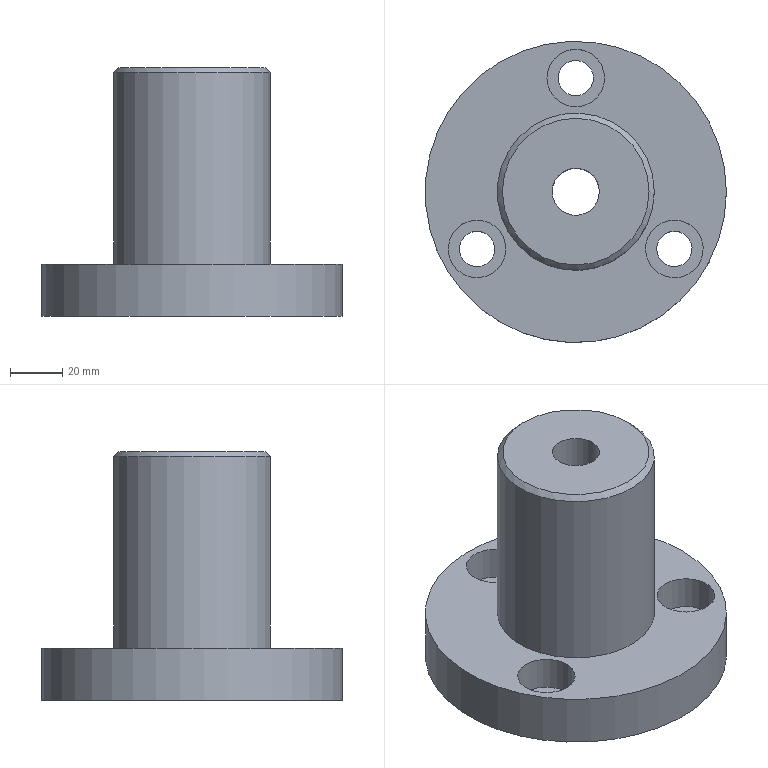Component | NX | DIE_SHANK | 1 solid | 16 faces | box 115 x 115 x 95 mm | volume 377421 mm3 | cylinder 9 | plane 6 | cone 1 | commonest cylinder face diameters 22 x3 13.5 x3 115 x1 60 x1 18 x1
STEP:
#1=CARTESIAN_POINT('',(0.,0.,0.));
#2=DIRECTION('',(0.,0.,1.));
#3=DIRECTION('',(1.,0.,0.));
#4=AXIS2_PLACEMENT_3D('',#1,#2,#3);
#5=CARTESIAN_POINT('',(43.172,-19.724,237.));
#6=VERTEX_POINT('',#5);
#7=CARTESIAN_POINT('',(37.672,-29.25,237.));
#8=DIRECTION('',(0.,0.,1.));
#9=DIRECTION('',(0.5,0.866,0.));
#10=AXIS2_PLACEMENT_3D('',#7,#8,#9);
#11=CIRCLE('',#10,11.);
#12=CARTESIAN_POINT('',(37.672,-29.25,250.));
#13=DIRECTION('',(0.,0.,-1.));
#14=DIRECTION('',(0.5,0.866,0.));
#15=AXIS2_PLACEMENT_3D('',#12,#13,#14);
#16=CYLINDRICAL_SURFACE('',#15,11.);
#17=CARTESIAN_POINT('',(6.283,13.));
#18=DIRECTION('',(-1.,0.));
#19=VECTOR('',#18,1.);
#20=LINE('',#17,#19);
#21=(GEOMETRIC_REPRESENTATION_CONTEXT(2)PARAMETRIC_REPRESENTATION_CONTEXT()REPRESENTATION_CONTEXT('',''));
#22=DEFINITIONAL_REPRESENTATION('',(#20),#21);
#23=PCURVE('',#16,#22);
#24=CARTESIAN_POINT('',(37.672,-29.25,237.));
#25=DIRECTION('',(0.,0.,-1.));
#26=DIRECTION('',(0.5,0.866,0.));
#27=AXIS2_PLACEMENT_3D('',#24,#25,#26);
#28=PLANE('',#27);
#29=CARTESIAN_POINT('',(11.,0.));
#30=CARTESIAN_POINT('',(11.,-19.053));
#31=CARTESIAN_POINT('',(-5.5,-9.526));
#32=CARTESIAN_POINT('',(-22.,-0.));
#33=CARTESIAN_POINT('',(-5.5,9.526));
#34=CARTESIAN_POINT('',(11.,19.053));
#35=CARTESIAN_POINT('',(11.,0.));
#36=(BOUNDED_CURVE()B_SPLINE_CURVE(2,(#29,#30,#31,#32,#33,#34,#35),.UNSPECIFIED.,.T.,.F.)B_SPLINE_CURVE_WITH_KNOTS((1,2,2,2,2,1),(-2.094,0.,2.094,4.189,6.283,8.378),.UNSPECIFIED.)CURVE()GEOMETRIC_REPRESENTATION_ITEM()RATIONAL_B_SPLINE_CURVE((1.,0.5,1.,0.5,1.,0.5,1.))REPRESENTATION_ITEM(''));
#37=(GEOMETRIC_REPRESENTATION_CONTEXT(2)PARAMETRIC_REPRESENTATION_CONTEXT()REPRESENTATION_CONTEXT('',''));
#38=DEFINITIONAL_REPRESENTATION('',(#36),#37);
#39=PCURVE('',#28,#38);
#40=SURFACE_CURVE('',#11,(#23,#39),.PCURVE_S1.);
#41=EDGE_CURVE('',#6,#6,#40,.T.);
#42=ORIENTED_EDGE('',*,*,#41,.T.);
#43=CARTESIAN_POINT('',(43.172,-19.724,250.));
#44=VERTEX_POINT('',#43);
#45=CARTESIAN_POINT('',(43.172,-19.724,250.));
#46=CARTESIAN_POINT('',(43.172,-19.724,237.));
#47=B_SPLINE_CURVE_WITH_KNOTS('',1,(#45,#46),.UNSPECIFIED.,.F.,.F.,(2,2),(0.,13.),.PIECEWISE_BEZIER_KNOTS.);
#48=CARTESIAN_POINT('',(0.,0.));
#49=DIRECTION('',(0.,1.));
#50=VECTOR('',#49,1.);
#51=LINE('',#48,#50);
#52=(GEOMETRIC_REPRESENTATION_CONTEXT(2)PARAMETRIC_REPRESENTATION_CONTEXT()REPRESENTATION_CONTEXT('',''));
#53=DEFINITIONAL_REPRESENTATION('',(#51),#52);
#54=PCURVE('',#16,#53);
#55=CARTESIAN_POINT('',(6.283,0.));
#56=DIRECTION('',(0.,1.));
#57=VECTOR('',#56,1.);
#58=LINE('',#55,#57);
#59=(GEOMETRIC_REPRESENTATION_CONTEXT(2)PARAMETRIC_REPRESENTATION_CONTEXT()REPRESENTATION_CONTEXT('',''));
#60=DEFINITIONAL_REPRESENTATION('',(#58),#59);
#61=PCURVE('',#16,#60);
#62=SEAM_CURVE('',#47,(#54,#61),.PCURVE_S1.);
#63=EDGE_CURVE('',#44,#6,#62,.T.);
#64=ORIENTED_EDGE('',*,*,#63,.F.);
#65=CARTESIAN_POINT('',(37.672,-29.25,250.));
#66=DIRECTION('',(0.,0.,-1.));
#67=DIRECTION('',(0.5,0.866,0.));
#68=AXIS2_PLACEMENT_3D('',#65,#66,#67);
#69=CIRCLE('',#68,11.);
#70=CARTESIAN_POINT('',(0.,0.));
#71=DIRECTION('',(1.,0.));
#72=VECTOR('',#71,1.);
#73=LINE('',#70,#72);
#74=(GEOMETRIC_REPRESENTATION_CONTEXT(2)PARAMETRIC_REPRESENTATION_CONTEXT()REPRESENTATION_CONTEXT('',''));
#75=DEFINITIONAL_REPRESENTATION('',(#73),#74);
#76=PCURVE('',#16,#75);
#77=CARTESIAN_POINT('',(-0.,-7.5,250.));
#78=DIRECTION('',(0.,0.,1.));
#79=DIRECTION('',(1.,0.,0.));
#80=AXIS2_PLACEMENT_3D('',#77,#78,#79);
#81=PLANE('',#80);
#82=CARTESIAN_POINT('',(43.172,-12.224));
#83=CARTESIAN_POINT('',(59.672,-21.75));
#84=CARTESIAN_POINT('',(43.172,-31.276));
#85=CARTESIAN_POINT('',(26.672,-40.803));
#86=CARTESIAN_POINT('',(26.672,-21.75));
#87=CARTESIAN_POINT('',(26.672,-2.697));
#88=CARTESIAN_POINT('',(43.172,-12.224));
#89=(BOUNDED_CURVE()B_SPLINE_CURVE(2,(#82,#83,#84,#85,#86,#87,#88),.UNSPECIFIED.,.T.,.F.)B_SPLINE_CURVE_WITH_KNOTS((1,2,2,2,2,1),(-2.094,0.,2.094,4.189,6.283,8.378),.UNSPECIFIED.)CURVE()GEOMETRIC_REPRESENTATION_ITEM()RATIONAL_B_SPLINE_CURVE((1.,0.5,1.,0.5,1.,0.5,1.))REPRESENTATION_ITEM(''));
#90=(GEOMETRIC_REPRESENTATION_CONTEXT(2)PARAMETRIC_REPRESENTATION_CONTEXT()REPRESENTATION_CONTEXT('',''));
#91=DEFINITIONAL_REPRESENTATION('',(#89),#90);
#92=PCURVE('',#81,#91);
#93=SURFACE_CURVE('',#69,(#76,#92),.PCURVE_S1.);
#94=EDGE_CURVE('',#44,#44,#93,.T.);
#95=ORIENTED_EDGE('',*,*,#94,.T.);
#96=ORIENTED_EDGE('',*,*,#63,.T.);
#97=EDGE_LOOP('',(#42,#64,#95,#96));
#98=FACE_BOUND('',#97,.F.);
#99=ADVANCED_FACE('',(#98),#16,.F.);
#100=CARTESIAN_POINT('',(41.047,-23.404,237.));
#101=VERTEX_POINT('',#100);
#102=CARTESIAN_POINT('',(37.672,-29.25,237.));
#103=DIRECTION('',(0.,0.,1.));
#104=DIRECTION('',(0.5,0.866,0.));
#105=AXIS2_PLACEMENT_3D('',#102,#103,#104);
#106=CIRCLE('',#105,6.75);
#107=CARTESIAN_POINT('',(6.75,0.));
#108=CARTESIAN_POINT('',(6.75,-11.691));
#109=CARTESIAN_POINT('',(-3.375,-5.846));
#110=CARTESIAN_POINT('',(-13.5,-0.));
#111=CARTESIAN_POINT('',(-3.375,5.846));
#112=CARTESIAN_POINT('',(6.75,11.691));
#113=CARTESIAN_POINT('',(6.75,0.));
#114=(BOUNDED_CURVE()B_SPLINE_CURVE(2,(#107,#108,#109,#110,#111,#112,#113),.UNSPECIFIED.,.T.,.F.)B_SPLINE_CURVE_WITH_KNOTS((1,2,2,2,2,1),(-2.094,0.,2.094,4.189,6.283,8.378),.UNSPECIFIED.)CURVE()GEOMETRIC_REPRESENTATION_ITEM()RATIONAL_B_SPLINE_CURVE((1.,0.5,1.,0.5,1.,0.5,1.))REPRESENTATION_ITEM(''));
#115=(GEOMETRIC_REPRESENTATION_CONTEXT(2)PARAMETRIC_REPRESENTATION_CONTEXT()REPRESENTATION_CONTEXT('',''));
#116=DEFINITIONAL_REPRESENTATION('',(#114),#115);
#117=PCURVE('',#28,#116);
#118=CARTESIAN_POINT('',(37.672,-29.25,183.484));
#119=DIRECTION('',(0.,0.,-1.));
#120=DIRECTION('',(0.5,0.866,0.));
#121=AXIS2_PLACEMENT_3D('',#118,#119,#120);
#122=CYLINDRICAL_SURFACE('',#121,6.75);
#123=CARTESIAN_POINT('',(6.283,-53.516));
#124=DIRECTION('',(-1.,0.));
#125=VECTOR('',#124,1.);
#126=LINE('',#123,#125);
#127=(GEOMETRIC_REPRESENTATION_CONTEXT(2)PARAMETRIC_REPRESENTATION_CONTEXT()REPRESENTATION_CONTEXT('',''));
#128=DEFINITIONAL_REPRESENTATION('',(#126),#127);
#129=PCURVE('',#122,#128);
#130=SURFACE_CURVE('',#106,(#117,#129),.PCURVE_S1.);
#131=EDGE_CURVE('',#101,#101,#130,.T.);
#132=ORIENTED_EDGE('',*,*,#131,.F.);
#133=EDGE_LOOP('',(#132));
#134=FACE_BOUND('',#133,.T.);
#135=ORIENTED_EDGE('',*,*,#41,.T.);
#136=EDGE_LOOP('',(#135));
#137=FACE_BOUND('',#136,.T.);
#138=ADVANCED_FACE('',(#134,#137),#28,.F.);
#139=CARTESIAN_POINT('',(41.047,-23.404,230.));
#140=VERTEX_POINT('',#139);
#141=CARTESIAN_POINT('',(37.672,-29.25,230.));
#142=DIRECTION('',(0.,0.,-1.));
#143=DIRECTION('',(0.5,0.866,0.));
#144=AXIS2_PLACEMENT_3D('',#141,#142,#143);
#145=CIRCLE('',#144,6.75);
#146=CARTESIAN_POINT('',(0.,-46.516));
#147=DIRECTION('',(1.,0.));
#148=VECTOR('',#147,1.);
#149=LINE('',#146,#148);
#150=(GEOMETRIC_REPRESENTATION_CONTEXT(2)PARAMETRIC_REPRESENTATION_CONTEXT()REPRESENTATION_CONTEXT('',''));
#151=DEFINITIONAL_REPRESENTATION('',(#149),#150);
#152=PCURVE('',#122,#151);
#153=CARTESIAN_POINT('',(-0.,-7.5,230.));
#154=DIRECTION('',(0.,0.,-1.));
#155=DIRECTION('',(-1.,0.,0.));
#156=AXIS2_PLACEMENT_3D('',#153,#154,#155);
#157=PLANE('',#156);
#158=CARTESIAN_POINT('',(-37.672,-21.75));
#159=DIRECTION('',(-0.5,0.866));
#160=AXIS2_PLACEMENT_2D('',#158,#159);
#161=CIRCLE('',#160,6.75);
#162=(GEOMETRIC_REPRESENTATION_CONTEXT(2)PARAMETRIC_REPRESENTATION_CONTEXT()REPRESENTATION_CONTEXT('',''));
#163=DEFINITIONAL_REPRESENTATION('',(#161),#162);
#164=PCURVE('',#157,#163);
#165=SURFACE_CURVE('',#145,(#152,#164),.PCURVE_S1.);
#166=EDGE_CURVE('',#140,#140,#165,.T.);
#167=ORIENTED_EDGE('',*,*,#166,.F.);
#168=CARTESIAN_POINT('',(41.047,-23.404,237.));
#169=CARTESIAN_POINT('',(41.047,-23.404,230.));
#170=B_SPLINE_CURVE_WITH_KNOTS('',1,(#168,#169),.UNSPECIFIED.,.F.,.F.,(2,2),(-53.516,-46.516),.PIECEWISE_BEZIER_KNOTS.);
#171=CARTESIAN_POINT('',(0.,0.));
#172=DIRECTION('',(0.,1.));
#173=VECTOR('',#172,1.);
#174=LINE('',#171,#173);
#175=(GEOMETRIC_REPRESENTATION_CONTEXT(2)PARAMETRIC_REPRESENTATION_CONTEXT()REPRESENTATION_CONTEXT('',''));
#176=DEFINITIONAL_REPRESENTATION('',(#174),#175);
#177=PCURVE('',#122,#176);
#178=CARTESIAN_POINT('',(6.283,0.));
#179=DIRECTION('',(0.,1.));
#180=VECTOR('',#179,1.);
#181=LINE('',#178,#180);
#182=(GEOMETRIC_REPRESENTATION_CONTEXT(2)PARAMETRIC_REPRESENTATION_CONTEXT()REPRESENTATION_CONTEXT('',''));
#183=DEFINITIONAL_REPRESENTATION('',(#181),#182);
#184=PCURVE('',#122,#183);
#185=SEAM_CURVE('',#170,(#177,#184),.PCURVE_S1.);
#186=EDGE_CURVE('',#101,#140,#185,.T.);
#187=ORIENTED_EDGE('',*,*,#186,.F.);
#188=ORIENTED_EDGE('',*,*,#131,.F.);
#189=ORIENTED_EDGE('',*,*,#186,.T.);
#190=EDGE_LOOP('',(#167,#187,#188,#189));
#191=FACE_BOUND('',#190,.F.);
#192=ADVANCED_FACE('',(#191),#122,.F.);
#193=CARTESIAN_POINT('',(-32.172,-38.776,237.));
#194=VERTEX_POINT('',#193);
#195=CARTESIAN_POINT('',(-37.672,-29.25,237.));
#196=DIRECTION('',(0.,0.,1.));
#197=DIRECTION('',(0.5,-0.866,0.));
#198=AXIS2_PLACEMENT_3D('',#195,#196,#197);
#199=CIRCLE('',#198,11.);
#200=CARTESIAN_POINT('',(-37.672,-29.25,250.));
#201=DIRECTION('',(0.,0.,-1.));
#202=DIRECTION('',(0.5,-0.866,0.));
#203=AXIS2_PLACEMENT_3D('',#200,#201,#202);
#204=CYLINDRICAL_SURFACE('',#203,11.);
#205=CARTESIAN_POINT('',(6.283,13.));
#206=DIRECTION('',(-1.,0.));
#207=VECTOR('',#206,1.);
#208=LINE('',#205,#207);
#209=(GEOMETRIC_REPRESENTATION_CONTEXT(2)PARAMETRIC_REPRESENTATION_CONTEXT()REPRESENTATION_CONTEXT('',''));
#210=DEFINITIONAL_REPRESENTATION('',(#208),#209);
#211=PCURVE('',#204,#210);
#212=CARTESIAN_POINT('',(-37.672,-29.25,237.));
#213=DIRECTION('',(0.,0.,-1.));
#214=DIRECTION('',(0.5,-0.866,0.));
#215=AXIS2_PLACEMENT_3D('',#212,#213,#214);
#216=PLANE('',#215);
#217=CARTESIAN_POINT('',(11.,0.));
#218=CARTESIAN_POINT('',(11.,-19.053));
#219=CARTESIAN_POINT('',(-5.5,-9.526));
#220=CARTESIAN_POINT('',(-22.,-0.));
#221=CARTESIAN_POINT('',(-5.5,9.526));
#222=CARTESIAN_POINT('',(11.,19.053));
#223=CARTESIAN_POINT('',(11.,0.));
#224=(BOUNDED_CURVE()B_SPLINE_CURVE(2,(#217,#218,#219,#220,#221,#222,#223),.UNSPECIFIED.,.T.,.F.)B_SPLINE_CURVE_WITH_KNOTS((1,2,2,2,2,1),(-2.094,0.,2.094,4.189,6.283,8.378),.UNSPECIFIED.)CURVE()GEOMETRIC_REPRESENTATION_ITEM()RATIONAL_B_SPLINE_CURVE((1.,0.5,1.,0.5,1.,0.5,1.))REPRESENTATION_ITEM(''));
#225=(GEOMETRIC_REPRESENTATION_CONTEXT(2)PARAMETRIC_REPRESENTATION_CONTEXT()REPRESENTATION_CONTEXT('',''));
#226=DEFINITIONAL_REPRESENTATION('',(#224),#225);
#227=PCURVE('',#216,#226);
#228=SURFACE_CURVE('',#199,(#211,#227),.PCURVE_S1.);
#229=EDGE_CURVE('',#194,#194,#228,.T.);
#230=ORIENTED_EDGE('',*,*,#229,.T.);
#231=CARTESIAN_POINT('',(-32.172,-38.776,250.));
#232=VERTEX_POINT('',#231);
#233=CARTESIAN_POINT('',(-32.172,-38.776,250.));
#234=CARTESIAN_POINT('',(-32.172,-38.776,237.));
#235=B_SPLINE_CURVE_WITH_KNOTS('',1,(#233,#234),.UNSPECIFIED.,.F.,.F.,(2,2),(0.,13.),.PIECEWISE_BEZIER_KNOTS.);
#236=CARTESIAN_POINT('',(0.,0.));
#237=DIRECTION('',(0.,1.));
#238=VECTOR('',#237,1.);
#239=LINE('',#236,#238);
#240=(GEOMETRIC_REPRESENTATION_CONTEXT(2)PARAMETRIC_REPRESENTATION_CONTEXT()REPRESENTATION_CONTEXT('',''));
#241=DEFINITIONAL_REPRESENTATION('',(#239),#240);
#242=PCURVE('',#204,#241);
#243=CARTESIAN_POINT('',(6.283,0.));
#244=DIRECTION('',(0.,1.));
#245=VECTOR('',#244,1.);
#246=LINE('',#243,#245);
#247=(GEOMETRIC_REPRESENTATION_CONTEXT(2)PARAMETRIC_REPRESENTATION_CONTEXT()REPRESENTATION_CONTEXT('',''));
#248=DEFINITIONAL_REPRESENTATION('',(#246),#247);
#249=PCURVE('',#204,#248);
#250=SEAM_CURVE('',#235,(#242,#249),.PCURVE_S1.);
#251=EDGE_CURVE('',#232,#194,#250,.T.);
#252=ORIENTED_EDGE('',*,*,#251,.F.);
#253=CARTESIAN_POINT('',(-37.672,-29.25,250.));
#254=DIRECTION('',(0.,0.,-1.));
#255=DIRECTION('',(0.5,-0.866,0.));
#256=AXIS2_PLACEMENT_3D('',#253,#254,#255);
#257=CIRCLE('',#256,11.);
#258=CARTESIAN_POINT('',(0.,0.));
#259=DIRECTION('',(1.,0.));
#260=VECTOR('',#259,1.);
#261=LINE('',#258,#260);
#262=(GEOMETRIC_REPRESENTATION_CONTEXT(2)PARAMETRIC_REPRESENTATION_CONTEXT()REPRESENTATION_CONTEXT('',''));
#263=DEFINITIONAL_REPRESENTATION('',(#261),#262);
#264=PCURVE('',#204,#263);
#265=CARTESIAN_POINT('',(-32.172,-31.276));
#266=CARTESIAN_POINT('',(-48.672,-40.803));
#267=CARTESIAN_POINT('',(-48.672,-21.75));
#268=CARTESIAN_POINT('',(-48.672,-2.697));
#269=CARTESIAN_POINT('',(-32.172,-12.224));
#270=CARTESIAN_POINT('',(-15.672,-21.75));
#271=CARTESIAN_POINT('',(-32.172,-31.276));
#272=(BOUNDED_CURVE()B_SPLINE_CURVE(2,(#265,#266,#267,#268,#269,#270,#271),.UNSPECIFIED.,.T.,.F.)B_SPLINE_CURVE_WITH_KNOTS((1,2,2,2,2,1),(-2.094,0.,2.094,4.189,6.283,8.378),.UNSPECIFIED.)CURVE()GEOMETRIC_REPRESENTATION_ITEM()RATIONAL_B_SPLINE_CURVE((1.,0.5,1.,0.5,1.,0.5,1.))REPRESENTATION_ITEM(''));
#273=(GEOMETRIC_REPRESENTATION_CONTEXT(2)PARAMETRIC_REPRESENTATION_CONTEXT()REPRESENTATION_CONTEXT('',''));
#274=DEFINITIONAL_REPRESENTATION('',(#272),#273);
#275=PCURVE('',#81,#274);
#276=SURFACE_CURVE('',#257,(#264,#275),.PCURVE_S1.);
#277=EDGE_CURVE('',#232,#232,#276,.T.);
#278=ORIENTED_EDGE('',*,*,#277,.T.);
#279=ORIENTED_EDGE('',*,*,#251,.T.);
#280=EDGE_LOOP('',(#230,#252,#278,#279));
#281=FACE_BOUND('',#280,.F.);
#282=ADVANCED_FACE('',(#281),#204,.F.);
#283=CARTESIAN_POINT('',(-34.297,-35.096,237.));
#284=VERTEX_POINT('',#283);
#285=CARTESIAN_POINT('',(-37.672,-29.25,237.));
#286=DIRECTION('',(0.,0.,1.));
#287=DIRECTION('',(0.5,-0.866,0.));
#288=AXIS2_PLACEMENT_3D('',#285,#286,#287);
#289=CIRCLE('',#288,6.75);
#290=CARTESIAN_POINT('',(6.75,0.));
#291=CARTESIAN_POINT('',(6.75,-11.691));
#292=CARTESIAN_POINT('',(-3.375,-5.846));
#293=CARTESIAN_POINT('',(-13.5,-0.));
#294=CARTESIAN_POINT('',(-3.375,5.846));
#295=CARTESIAN_POINT('',(6.75,11.691));
#296=CARTESIAN_POINT('',(6.75,0.));
#297=(BOUNDED_CURVE()B_SPLINE_CURVE(2,(#290,#291,#292,#293,#294,#295,#296),.UNSPECIFIED.,.T.,.F.)B_SPLINE_CURVE_WITH_KNOTS((1,2,2,2,2,1),(-2.094,0.,2.094,4.189,6.283,8.378),.UNSPECIFIED.)CURVE()GEOMETRIC_REPRESENTATION_ITEM()RATIONAL_B_SPLINE_CURVE((1.,0.5,1.,0.5,1.,0.5,1.))REPRESENTATION_ITEM(''));
#298=(GEOMETRIC_REPRESENTATION_CONTEXT(2)PARAMETRIC_REPRESENTATION_CONTEXT()REPRESENTATION_CONTEXT('',''));
#299=DEFINITIONAL_REPRESENTATION('',(#297),#298);
#300=PCURVE('',#216,#299);
#301=CARTESIAN_POINT('',(-37.672,-29.25,183.484));
#302=DIRECTION('',(0.,0.,-1.));
#303=DIRECTION('',(0.5,-0.866,0.));
#304=AXIS2_PLACEMENT_3D('',#301,#302,#303);
#305=CYLINDRICAL_SURFACE('',#304,6.75);
#306=CARTESIAN_POINT('',(6.283,-53.516));
#307=DIRECTION('',(-1.,0.));
#308=VECTOR('',#307,1.);
#309=LINE('',#306,#308);
#310=(GEOMETRIC_REPRESENTATION_CONTEXT(2)PARAMETRIC_REPRESENTATION_CONTEXT()REPRESENTATION_CONTEXT('',''));
#311=DEFINITIONAL_REPRESENTATION('',(#309),#310);
#312=PCURVE('',#305,#311);
#313=SURFACE_CURVE('',#289,(#300,#312),.PCURVE_S1.);
#314=EDGE_CURVE('',#284,#284,#313,.T.);
#315=ORIENTED_EDGE('',*,*,#314,.F.);
#316=EDGE_LOOP('',(#315));
#317=FACE_BOUND('',#316,.T.);
#318=ORIENTED_EDGE('',*,*,#229,.T.);
#319=EDGE_LOOP('',(#318));
#320=FACE_BOUND('',#319,.T.);
#321=ADVANCED_FACE('',(#317,#320),#216,.F.);
#322=CARTESIAN_POINT('',(-34.297,-35.096,230.));
#323=VERTEX_POINT('',#322);
#324=CARTESIAN_POINT('',(-37.672,-29.25,230.));
#325=DIRECTION('',(0.,0.,-1.));
#326=DIRECTION('',(0.5,-0.866,0.));
#327=AXIS2_PLACEMENT_3D('',#324,#325,#326);
#328=CIRCLE('',#327,6.75);
#329=CARTESIAN_POINT('',(0.,-46.516));
#330=DIRECTION('',(1.,0.));
#331=VECTOR('',#330,1.);
#332=LINE('',#329,#331);
#333=(GEOMETRIC_REPRESENTATION_CONTEXT(2)PARAMETRIC_REPRESENTATION_CONTEXT()REPRESENTATION_CONTEXT('',''));
#334=DEFINITIONAL_REPRESENTATION('',(#332),#333);
#335=PCURVE('',#305,#334);
#336=CARTESIAN_POINT('',(37.672,-21.75));
#337=DIRECTION('',(-0.5,-0.866));
#338=AXIS2_PLACEMENT_2D('',#336,#337);
#339=CIRCLE('',#338,6.75);
#340=(GEOMETRIC_REPRESENTATION_CONTEXT(2)PARAMETRIC_REPRESENTATION_CONTEXT()REPRESENTATION_CONTEXT('',''));
#341=DEFINITIONAL_REPRESENTATION('',(#339),#340);
#342=PCURVE('',#157,#341);
#343=SURFACE_CURVE('',#328,(#335,#342),.PCURVE_S1.);
#344=EDGE_CURVE('',#323,#323,#343,.T.);
#345=ORIENTED_EDGE('',*,*,#344,.F.);
#346=CARTESIAN_POINT('',(-34.297,-35.096,237.));
#347=CARTESIAN_POINT('',(-34.297,-35.096,230.));
#348=B_SPLINE_CURVE_WITH_KNOTS('',1,(#346,#347),.UNSPECIFIED.,.F.,.F.,(2,2),(-53.516,-46.516),.PIECEWISE_BEZIER_KNOTS.);
#349=CARTESIAN_POINT('',(0.,0.));
#350=DIRECTION('',(0.,1.));
#351=VECTOR('',#350,1.);
#352=LINE('',#349,#351);
#353=(GEOMETRIC_REPRESENTATION_CONTEXT(2)PARAMETRIC_REPRESENTATION_CONTEXT()REPRESENTATION_CONTEXT('',''));
#354=DEFINITIONAL_REPRESENTATION('',(#352),#353);
#355=PCURVE('',#305,#354);
#356=CARTESIAN_POINT('',(6.283,0.));
#357=DIRECTION('',(0.,1.));
#358=VECTOR('',#357,1.);
#359=LINE('',#356,#358);
#360=(GEOMETRIC_REPRESENTATION_CONTEXT(2)PARAMETRIC_REPRESENTATION_CONTEXT()REPRESENTATION_CONTEXT('',''));
#361=DEFINITIONAL_REPRESENTATION('',(#359),#360);
#362=PCURVE('',#305,#361);
#363=SEAM_CURVE('',#348,(#355,#362),.PCURVE_S1.);
#364=EDGE_CURVE('',#284,#323,#363,.T.);
#365=ORIENTED_EDGE('',*,*,#364,.F.);
#366=ORIENTED_EDGE('',*,*,#314,.F.);
#367=ORIENTED_EDGE('',*,*,#364,.T.);
#368=EDGE_LOOP('',(#345,#365,#366,#367));
#369=FACE_BOUND('',#368,.F.);
#370=ADVANCED_FACE('',(#369),#305,.F.);
#371=ORIENTED_EDGE('',*,*,#94,.T.);
#372=EDGE_LOOP('',(#371));
#373=FACE_BOUND('',#372,.T.);
#374=ORIENTED_EDGE('',*,*,#277,.T.);
#375=EDGE_LOOP('',(#374));
#376=FACE_BOUND('',#375,.T.);
#377=CARTESIAN_POINT('',(-11.,36.,250.));
#378=VERTEX_POINT('',#377);
#379=CARTESIAN_POINT('',(-0.,36.,250.));
#380=DIRECTION('',(0.,0.,-1.));
#381=DIRECTION('',(-1.,0.,0.));
#382=AXIS2_PLACEMENT_3D('',#379,#380,#381);
#383=CIRCLE('',#382,11.);
#384=CARTESIAN_POINT('',(-11.,43.5));
#385=CARTESIAN_POINT('',(-11.,62.553));
#386=CARTESIAN_POINT('',(5.5,53.026));
#387=CARTESIAN_POINT('',(22.,43.5));
#388=CARTESIAN_POINT('',(5.5,33.974));
#389=CARTESIAN_POINT('',(-11.,24.447));
#390=CARTESIAN_POINT('',(-11.,43.5));
#391=(BOUNDED_CURVE()B_SPLINE_CURVE(2,(#384,#385,#386,#387,#388,#389,#390),.UNSPECIFIED.,.T.,.F.)B_SPLINE_CURVE_WITH_KNOTS((1,2,2,2,2,1),(-2.094,0.,2.094,4.189,6.283,8.378),.UNSPECIFIED.)CURVE()GEOMETRIC_REPRESENTATION_ITEM()RATIONAL_B_SPLINE_CURVE((1.,0.5,1.,0.5,1.,0.5,1.))REPRESENTATION_ITEM(''));
#392=(GEOMETRIC_REPRESENTATION_CONTEXT(2)PARAMETRIC_REPRESENTATION_CONTEXT()REPRESENTATION_CONTEXT('',''));
#393=DEFINITIONAL_REPRESENTATION('',(#391),#392);
#394=PCURVE('',#81,#393);
#395=CARTESIAN_POINT('',(-0.,36.,250.));
#396=DIRECTION('',(0.,0.,-1.));
#397=DIRECTION('',(-1.,0.,0.));
#398=AXIS2_PLACEMENT_3D('',#395,#396,#397);
#399=CYLINDRICAL_SURFACE('',#398,11.);
#400=CARTESIAN_POINT('',(0.,0.));
#401=DIRECTION('',(1.,0.));
#402=VECTOR('',#401,1.);
#403=LINE('',#400,#402);
#404=(GEOMETRIC_REPRESENTATION_CONTEXT(2)PARAMETRIC_REPRESENTATION_CONTEXT()REPRESENTATION_CONTEXT('',''));
#405=DEFINITIONAL_REPRESENTATION('',(#403),#404);
#406=PCURVE('',#399,#405);
#407=SURFACE_CURVE('',#383,(#394,#406),.PCURVE_S1.);
#408=EDGE_CURVE('',#378,#378,#407,.T.);
#409=ORIENTED_EDGE('',*,*,#408,.T.);
#410=EDGE_LOOP('',(#409));
#411=FACE_BOUND('',#410,.T.);
#412=CARTESIAN_POINT('',(30.,-7.5,250.));
#413=VERTEX_POINT('',#412);
#414=CARTESIAN_POINT('',(-0.,-7.5,250.));
#415=DIRECTION('',(0.,0.,1.));
#416=DIRECTION('',(1.,0.,0.));
#417=AXIS2_PLACEMENT_3D('',#414,#415,#416);
#418=CIRCLE('',#417,30.);
#419=CARTESIAN_POINT('',(0.,0.));
#420=DIRECTION('',(1.,0.));
#421=AXIS2_PLACEMENT_2D('',#419,#420);
#422=CIRCLE('',#421,30.);
#423=(GEOMETRIC_REPRESENTATION_CONTEXT(2)PARAMETRIC_REPRESENTATION_CONTEXT()REPRESENTATION_CONTEXT('',''));
#424=DEFINITIONAL_REPRESENTATION('',(#422),#423);
#425=PCURVE('',#81,#424);
#426=CARTESIAN_POINT('',(-0.,-7.5,250.));
#427=DIRECTION('',(0.,0.,1.));
#428=DIRECTION('',(1.,0.,0.));
#429=AXIS2_PLACEMENT_3D('',#426,#427,#428);
#430=CYLINDRICAL_SURFACE('',#429,30.);
#431=CARTESIAN_POINT('',(0.,0.));
#432=DIRECTION('',(1.,0.));
#433=VECTOR('',#432,1.);
#434=LINE('',#431,#433);
#435=(GEOMETRIC_REPRESENTATION_CONTEXT(2)PARAMETRIC_REPRESENTATION_CONTEXT()REPRESENTATION_CONTEXT('',''));
#436=DEFINITIONAL_REPRESENTATION('',(#434),#435);
#437=PCURVE('',#430,#436);
#438=SURFACE_CURVE('',#418,(#425,#437),.PCURVE_S1.);
#439=EDGE_CURVE('',#413,#413,#438,.T.);
#440=ORIENTED_EDGE('',*,*,#439,.F.);
#441=EDGE_LOOP('',(#440));
#442=FACE_BOUND('',#441,.T.);
#443=CARTESIAN_POINT('',(57.5,-7.5,250.));
#444=VERTEX_POINT('',#443);
#445=CARTESIAN_POINT('',(-0.,-7.5,250.));
#446=DIRECTION('',(0.,0.,-1.));
#447=DIRECTION('',(1.,0.,0.));
#448=AXIS2_PLACEMENT_3D('',#445,#446,#447);
#449=CIRCLE('',#448,57.5);
#450=CARTESIAN_POINT('',(57.5,0.));
#451=CARTESIAN_POINT('',(57.5,-99.593));
#452=CARTESIAN_POINT('',(-28.75,-49.796));
#453=CARTESIAN_POINT('',(-115.,-0.));
#454=CARTESIAN_POINT('',(-28.75,49.796));
#455=CARTESIAN_POINT('',(57.5,99.593));
#456=CARTESIAN_POINT('',(57.5,0.));
#457=(BOUNDED_CURVE()B_SPLINE_CURVE(2,(#450,#451,#452,#453,#454,#455,#456),.UNSPECIFIED.,.T.,.F.)B_SPLINE_CURVE_WITH_KNOTS((1,2,2,2,2,1),(-2.094,0.,2.094,4.189,6.283,8.378),.UNSPECIFIED.)CURVE()GEOMETRIC_REPRESENTATION_ITEM()RATIONAL_B_SPLINE_CURVE((1.,0.5,1.,0.5,1.,0.5,1.))REPRESENTATION_ITEM(''));
#458=(GEOMETRIC_REPRESENTATION_CONTEXT(2)PARAMETRIC_REPRESENTATION_CONTEXT()REPRESENTATION_CONTEXT('',''));
#459=DEFINITIONAL_REPRESENTATION('',(#457),#458);
#460=PCURVE('',#81,#459);
#461=CARTESIAN_POINT('',(-0.,-7.5,230.));
#462=DIRECTION('',(0.,0.,1.));
#463=DIRECTION('',(1.,0.,0.));
#464=AXIS2_PLACEMENT_3D('',#461,#462,#463);
#465=CYLINDRICAL_SURFACE('',#464,57.5);
#466=CARTESIAN_POINT('',(6.283,20.));
#467=DIRECTION('',(-1.,0.));
#468=VECTOR('',#467,1.);
#469=LINE('',#466,#468);
#470=(GEOMETRIC_REPRESENTATION_CONTEXT(2)PARAMETRIC_REPRESENTATION_CONTEXT()REPRESENTATION_CONTEXT('',''));
#471=DEFINITIONAL_REPRESENTATION('',(#469),#470);
#472=PCURVE('',#465,#471);
#473=SURFACE_CURVE('',#449,(#460,#472),.PCURVE_S1.);
#474=EDGE_CURVE('',#444,#444,#473,.T.);
#475=ORIENTED_EDGE('',*,*,#474,.F.);
#476=EDGE_LOOP('',(#475));
#477=FACE_BOUND('',#476,.T.);
#478=ADVANCED_FACE('',(#373,#376,#411,#442,#477),#81,.T.);
#479=ORIENTED_EDGE('',*,*,#166,.F.);
#480=EDGE_LOOP('',(#479));
#481=FACE_BOUND('',#480,.T.);
#482=ORIENTED_EDGE('',*,*,#344,.F.);
#483=EDGE_LOOP('',(#482));
#484=FACE_BOUND('',#483,.T.);
#485=CARTESIAN_POINT('',(-6.75,36.,230.));
#486=VERTEX_POINT('',#485);
#487=CARTESIAN_POINT('',(-0.,36.,230.));
#488=DIRECTION('',(0.,0.,-1.));
#489=DIRECTION('',(-1.,0.,0.));
#490=AXIS2_PLACEMENT_3D('',#487,#488,#489);
#491=CIRCLE('',#490,6.75);
#492=CARTESIAN_POINT('',(0.,43.5));
#493=DIRECTION('',(1.,0.));
#494=AXIS2_PLACEMENT_2D('',#492,#493);
#495=CIRCLE('',#494,6.75);
#496=(GEOMETRIC_REPRESENTATION_CONTEXT(2)PARAMETRIC_REPRESENTATION_CONTEXT()REPRESENTATION_CONTEXT('',''));
#497=DEFINITIONAL_REPRESENTATION('',(#495),#496);
#498=PCURVE('',#157,#497);
#499=CARTESIAN_POINT('',(-0.,36.,183.484));
#500=DIRECTION('',(0.,0.,-1.));
#501=DIRECTION('',(-1.,0.,0.));
#502=AXIS2_PLACEMENT_3D('',#499,#500,#501);
#503=CYLINDRICAL_SURFACE('',#502,6.75);
#504=CARTESIAN_POINT('',(0.,-46.516));
#505=DIRECTION('',(1.,0.));
#506=VECTOR('',#505,1.);
#507=LINE('',#504,#506);
#508=(GEOMETRIC_REPRESENTATION_CONTEXT(2)PARAMETRIC_REPRESENTATION_CONTEXT()REPRESENTATION_CONTEXT('',''));
#509=DEFINITIONAL_REPRESENTATION('',(#507),#508);
#510=PCURVE('',#503,#509);
#511=SURFACE_CURVE('',#491,(#498,#510),.PCURVE_S1.);
#512=EDGE_CURVE('',#486,#486,#511,.T.);
#513=ORIENTED_EDGE('',*,*,#512,.F.);
#514=EDGE_LOOP('',(#513));
#515=FACE_BOUND('',#514,.T.);
#516=CARTESIAN_POINT('',(-9.,-7.5,230.));
#517=VERTEX_POINT('',#516);
#518=CARTESIAN_POINT('',(-0.,-7.5,230.));
#519=DIRECTION('',(0.,0.,-1.));
#520=DIRECTION('',(-1.,0.,0.));
#521=AXIS2_PLACEMENT_3D('',#518,#519,#520);
#522=CIRCLE('',#521,9.);
#523=CARTESIAN_POINT('',(0.,0.));
#524=DIRECTION('',(1.,0.));
#525=AXIS2_PLACEMENT_2D('',#523,#524);
#526=CIRCLE('',#525,9.);
#527=(GEOMETRIC_REPRESENTATION_CONTEXT(2)PARAMETRIC_REPRESENTATION_CONTEXT()REPRESENTATION_CONTEXT('',''));
#528=DEFINITIONAL_REPRESENTATION('',(#526),#527);
#529=PCURVE('',#157,#528);
#530=CARTESIAN_POINT('',(-0.,-7.5,325.));
#531=DIRECTION('',(0.,0.,-1.));
#532=DIRECTION('',(-1.,0.,0.));
#533=AXIS2_PLACEMENT_3D('',#530,#531,#532);
#534=CYLINDRICAL_SURFACE('',#533,9.);
#535=CARTESIAN_POINT('',(0.,95.));
#536=DIRECTION('',(1.,0.));
#537=VECTOR('',#536,1.);
#538=LINE('',#535,#537);
#539=(GEOMETRIC_REPRESENTATION_CONTEXT(2)PARAMETRIC_REPRESENTATION_CONTEXT()REPRESENTATION_CONTEXT('',''));
#540=DEFINITIONAL_REPRESENTATION('',(#538),#539);
#541=PCURVE('',#534,#540);
#542=SURFACE_CURVE('',#522,(#529,#541),.PCURVE_S1.);
#543=EDGE_CURVE('',#517,#517,#542,.T.);
#544=ORIENTED_EDGE('',*,*,#543,.F.);
#545=EDGE_LOOP('',(#544));
#546=FACE_BOUND('',#545,.T.);
#547=CARTESIAN_POINT('',(57.5,-7.5,230.));
#548=VERTEX_POINT('',#547);
#549=CARTESIAN_POINT('',(-0.,-7.5,230.));
#550=DIRECTION('',(0.,0.,1.));
#551=DIRECTION('',(1.,0.,0.));
#552=AXIS2_PLACEMENT_3D('',#549,#550,#551);
#553=CIRCLE('',#552,57.5);
#554=CARTESIAN_POINT('',(-57.5,0.));
#555=CARTESIAN_POINT('',(-57.5,99.593));
#556=CARTESIAN_POINT('',(28.75,49.796));
#557=CARTESIAN_POINT('',(115.,0.));
#558=CARTESIAN_POINT('',(28.75,-49.796));
#559=CARTESIAN_POINT('',(-57.5,-99.593));
#560=CARTESIAN_POINT('',(-57.5,0.));
#561=(BOUNDED_CURVE()B_SPLINE_CURVE(2,(#554,#555,#556,#557,#558,#559,#560),.UNSPECIFIED.,.T.,.F.)B_SPLINE_CURVE_WITH_KNOTS((1,2,2,2,2,1),(-2.094,0.,2.094,4.189,6.283,8.378),.UNSPECIFIED.)CURVE()GEOMETRIC_REPRESENTATION_ITEM()RATIONAL_B_SPLINE_CURVE((1.,0.5,1.,0.5,1.,0.5,1.))REPRESENTATION_ITEM(''));
#562=(GEOMETRIC_REPRESENTATION_CONTEXT(2)PARAMETRIC_REPRESENTATION_CONTEXT()REPRESENTATION_CONTEXT('',''));
#563=DEFINITIONAL_REPRESENTATION('',(#561),#562);
#564=PCURVE('',#157,#563);
#565=CARTESIAN_POINT('',(0.,0.));
#566=DIRECTION('',(1.,0.));
#567=VECTOR('',#566,1.);
#568=LINE('',#565,#567);
#569=(GEOMETRIC_REPRESENTATION_CONTEXT(2)PARAMETRIC_REPRESENTATION_CONTEXT()REPRESENTATION_CONTEXT('',''));
#570=DEFINITIONAL_REPRESENTATION('',(#568),#569);
#571=PCURVE('',#465,#570);
#572=SURFACE_CURVE('',#553,(#564,#571),.PCURVE_S1.);
#573=EDGE_CURVE('',#548,#548,#572,.T.);
#574=ORIENTED_EDGE('',*,*,#573,.F.);
#575=EDGE_LOOP('',(#574));
#576=FACE_BOUND('',#575,.T.);
#577=ADVANCED_FACE('',(#481,#484,#515,#546,#576),#157,.T.);
#578=ORIENTED_EDGE('',*,*,#474,.T.);
#579=CARTESIAN_POINT('',(57.5,-7.5,230.));
#580=CARTESIAN_POINT('',(57.5,-7.5,250.));
#581=B_SPLINE_CURVE_WITH_KNOTS('',1,(#579,#580),.UNSPECIFIED.,.F.,.F.,(2,2),(0.,20.),.PIECEWISE_BEZIER_KNOTS.);
#582=CARTESIAN_POINT('',(0.,0.));
#583=DIRECTION('',(0.,1.));
#584=VECTOR('',#583,1.);
#585=LINE('',#582,#584);
#586=(GEOMETRIC_REPRESENTATION_CONTEXT(2)PARAMETRIC_REPRESENTATION_CONTEXT()REPRESENTATION_CONTEXT('',''));
#587=DEFINITIONAL_REPRESENTATION('',(#585),#586);
#588=PCURVE('',#465,#587);
#589=CARTESIAN_POINT('',(6.283,0.));
#590=DIRECTION('',(0.,1.));
#591=VECTOR('',#590,1.);
#592=LINE('',#589,#591);
#593=(GEOMETRIC_REPRESENTATION_CONTEXT(2)PARAMETRIC_REPRESENTATION_CONTEXT()REPRESENTATION_CONTEXT('',''));
#594=DEFINITIONAL_REPRESENTATION('',(#592),#593);
#595=PCURVE('',#465,#594);
#596=SEAM_CURVE('',#581,(#588,#595),.PCURVE_S1.);
#597=EDGE_CURVE('',#548,#444,#596,.T.);
#598=ORIENTED_EDGE('',*,*,#597,.F.);
#599=ORIENTED_EDGE('',*,*,#573,.T.);
#600=ORIENTED_EDGE('',*,*,#597,.T.);
#601=EDGE_LOOP('',(#578,#598,#599,#600));
#602=FACE_BOUND('',#601,.T.);
#603=ADVANCED_FACE('',(#602),#465,.T.);
#604=CARTESIAN_POINT('',(-9.,-7.5,325.));
#605=VERTEX_POINT('',#604);
#606=CARTESIAN_POINT('',(-0.,-7.5,325.));
#607=DIRECTION('',(0.,0.,-1.));
#608=DIRECTION('',(-1.,0.,0.));
#609=AXIS2_PLACEMENT_3D('',#606,#607,#608);
#610=CIRCLE('',#609,9.);
#611=CARTESIAN_POINT('',(-0.,-7.5,325.));
#612=DIRECTION('',(0.,0.,1.));
#613=DIRECTION('',(1.,0.,0.));
#614=AXIS2_PLACEMENT_3D('',#611,#612,#613);
#615=PLANE('',#614);
#616=CARTESIAN_POINT('',(-9.,0.));
#617=CARTESIAN_POINT('',(-9.,15.588));
#618=CARTESIAN_POINT('',(4.5,7.794));
#619=CARTESIAN_POINT('',(18.,0.));
#620=CARTESIAN_POINT('',(4.5,-7.794));
#621=CARTESIAN_POINT('',(-9.,-15.588));
#622=CARTESIAN_POINT('',(-9.,0.));
#623=(BOUNDED_CURVE()B_SPLINE_CURVE(2,(#616,#617,#618,#619,#620,#621,#622),.UNSPECIFIED.,.T.,.F.)B_SPLINE_CURVE_WITH_KNOTS((1,2,2,2,2,1),(-2.094,0.,2.094,4.189,6.283,8.378),.UNSPECIFIED.)CURVE()GEOMETRIC_REPRESENTATION_ITEM()RATIONAL_B_SPLINE_CURVE((1.,0.5,1.,0.5,1.,0.5,1.))REPRESENTATION_ITEM(''));
#624=(GEOMETRIC_REPRESENTATION_CONTEXT(2)PARAMETRIC_REPRESENTATION_CONTEXT()REPRESENTATION_CONTEXT('',''));
#625=DEFINITIONAL_REPRESENTATION('',(#623),#624);
#626=PCURVE('',#615,#625);
#627=CARTESIAN_POINT('',(0.,0.));
#628=DIRECTION('',(1.,0.));
#629=VECTOR('',#628,1.);
#630=LINE('',#627,#629);
#631=(GEOMETRIC_REPRESENTATION_CONTEXT(2)PARAMETRIC_REPRESENTATION_CONTEXT()REPRESENTATION_CONTEXT('',''));
#632=DEFINITIONAL_REPRESENTATION('',(#630),#631);
#633=PCURVE('',#534,#632);
#634=SURFACE_CURVE('',#610,(#626,#633),.PCURVE_S1.);
#635=EDGE_CURVE('',#605,#605,#634,.T.);
#636=ORIENTED_EDGE('',*,*,#635,.T.);
#637=EDGE_LOOP('',(#636));
#638=FACE_BOUND('',#637,.T.);
#639=CARTESIAN_POINT('',(28.,-7.5,325.));
#640=VERTEX_POINT('',#639);
#641=CARTESIAN_POINT('',(-0.,-7.5,325.));
#642=DIRECTION('',(0.,0.,1.));
#643=DIRECTION('',(1.,0.,0.));
#644=AXIS2_PLACEMENT_3D('',#641,#642,#643);
#645=CIRCLE('',#644,28.);
#646=CARTESIAN_POINT('',(0.,0.));
#647=DIRECTION('',(1.,0.));
#648=AXIS2_PLACEMENT_2D('',#646,#647);
#649=CIRCLE('',#648,28.);
#650=(GEOMETRIC_REPRESENTATION_CONTEXT(2)PARAMETRIC_REPRESENTATION_CONTEXT()REPRESENTATION_CONTEXT('',''));
#651=DEFINITIONAL_REPRESENTATION('',(#649),#650);
#652=PCURVE('',#615,#651);
#653=CARTESIAN_POINT('',(-0.,-7.5,323.));
#654=DIRECTION('',(0.,0.,-1.));
#655=DIRECTION('',(-1.,0.,0.));
#656=AXIS2_PLACEMENT_3D('',#653,#654,#655);
#657=CONICAL_SURFACE('',#656,30.,0.7854);
#658=CARTESIAN_POINT('',(9.425,-2.));
#659=DIRECTION('',(-1.,0.));
#660=VECTOR('',#659,1.);
#661=LINE('',#658,#660);
#662=(GEOMETRIC_REPRESENTATION_CONTEXT(2)PARAMETRIC_REPRESENTATION_CONTEXT()REPRESENTATION_CONTEXT('',''));
#663=DEFINITIONAL_REPRESENTATION('',(#661),#662);
#664=PCURVE('',#657,#663);
#665=SURFACE_CURVE('',#645,(#652,#664),.PCURVE_S1.);
#666=EDGE_CURVE('',#640,#640,#665,.T.);
#667=ORIENTED_EDGE('',*,*,#666,.T.);
#668=EDGE_LOOP('',(#667));
#669=FACE_BOUND('',#668,.T.);
#670=ADVANCED_FACE('',(#638,#669),#615,.T.);
#671=CARTESIAN_POINT('',(30.,-7.5,323.));
#672=VERTEX_POINT('',#671);
#673=CARTESIAN_POINT('',(-0.,-7.5,323.));
#674=DIRECTION('',(0.,0.,-1.));
#675=DIRECTION('',(1.,0.,0.));
#676=AXIS2_PLACEMENT_3D('',#673,#674,#675);
#677=CIRCLE('',#676,30.);
#678=CARTESIAN_POINT('',(6.283,73.));
#679=DIRECTION('',(-1.,0.));
#680=VECTOR('',#679,1.);
#681=LINE('',#678,#680);
#682=(GEOMETRIC_REPRESENTATION_CONTEXT(2)PARAMETRIC_REPRESENTATION_CONTEXT()REPRESENTATION_CONTEXT('',''));
#683=DEFINITIONAL_REPRESENTATION('',(#681),#682);
#684=PCURVE('',#430,#683);
#685=CARTESIAN_POINT('',(3.142,0.));
#686=DIRECTION('',(1.,0.));
#687=VECTOR('',#686,1.);
#688=LINE('',#685,#687);
#689=(GEOMETRIC_REPRESENTATION_CONTEXT(2)PARAMETRIC_REPRESENTATION_CONTEXT()REPRESENTATION_CONTEXT('',''));
#690=DEFINITIONAL_REPRESENTATION('',(#688),#689);
#691=PCURVE('',#657,#690);
#692=SURFACE_CURVE('',#677,(#684,#691),.PCURVE_S1.);
#693=EDGE_CURVE('',#672,#672,#692,.T.);
#694=ORIENTED_EDGE('',*,*,#693,.T.);
#695=CARTESIAN_POINT('',(30.,-7.5,250.));
#696=CARTESIAN_POINT('',(30.,-7.5,323.));
#697=B_SPLINE_CURVE_WITH_KNOTS('',1,(#695,#696),.UNSPECIFIED.,.F.,.F.,(2,2),(0.,73.),.PIECEWISE_BEZIER_KNOTS.);
#698=CARTESIAN_POINT('',(0.,0.));
#699=DIRECTION('',(0.,1.));
#700=VECTOR('',#699,1.);
#701=LINE('',#698,#700);
#702=(GEOMETRIC_REPRESENTATION_CONTEXT(2)PARAMETRIC_REPRESENTATION_CONTEXT()REPRESENTATION_CONTEXT('',''));
#703=DEFINITIONAL_REPRESENTATION('',(#701),#702);
#704=PCURVE('',#430,#703);
#705=CARTESIAN_POINT('',(6.283,0.));
#706=DIRECTION('',(0.,1.));
#707=VECTOR('',#706,1.);
#708=LINE('',#705,#707);
#709=(GEOMETRIC_REPRESENTATION_CONTEXT(2)PARAMETRIC_REPRESENTATION_CONTEXT()REPRESENTATION_CONTEXT('',''));
#710=DEFINITIONAL_REPRESENTATION('',(#708),#709);
#711=PCURVE('',#430,#710);
#712=SEAM_CURVE('',#697,(#704,#711),.PCURVE_S1.);
#713=EDGE_CURVE('',#413,#672,#712,.T.);
#714=ORIENTED_EDGE('',*,*,#713,.F.);
#715=ORIENTED_EDGE('',*,*,#439,.T.);
#716=ORIENTED_EDGE('',*,*,#713,.T.);
#717=EDGE_LOOP('',(#694,#714,#715,#716));
#718=FACE_BOUND('',#717,.T.);
#719=ADVANCED_FACE('',(#718),#430,.T.);
#720=ORIENTED_EDGE('',*,*,#666,.F.);
#721=CARTESIAN_POINT('',(28.,-7.5,325.));
#722=CARTESIAN_POINT('',(30.,-7.5,323.));
#723=B_SPLINE_CURVE_WITH_KNOTS('',1,(#721,#722),.UNSPECIFIED.,.F.,.F.,(2,2),(-2.828,0.),.PIECEWISE_BEZIER_KNOTS.);
#724=CARTESIAN_POINT('',(9.425,0.));
#725=DIRECTION('',(0.,1.));
#726=VECTOR('',#725,1.);
#727=LINE('',#724,#726);
#728=(GEOMETRIC_REPRESENTATION_CONTEXT(2)PARAMETRIC_REPRESENTATION_CONTEXT()REPRESENTATION_CONTEXT('',''));
#729=DEFINITIONAL_REPRESENTATION('',(#727),#728);
#730=PCURVE('',#657,#729);
#731=CARTESIAN_POINT('',(3.142,0.));
#732=DIRECTION('',(0.,1.));
#733=VECTOR('',#732,1.);
#734=LINE('',#731,#733);
#735=(GEOMETRIC_REPRESENTATION_CONTEXT(2)PARAMETRIC_REPRESENTATION_CONTEXT()REPRESENTATION_CONTEXT('',''));
#736=DEFINITIONAL_REPRESENTATION('',(#734),#735);
#737=PCURVE('',#657,#736);
#738=SEAM_CURVE('',#723,(#730,#737),.PCURVE_S1.);
#739=EDGE_CURVE('',#640,#672,#738,.T.);
#740=ORIENTED_EDGE('',*,*,#739,.T.);
#741=ORIENTED_EDGE('',*,*,#693,.F.);
#742=ORIENTED_EDGE('',*,*,#739,.F.);
#743=EDGE_LOOP('',(#720,#740,#741,#742));
#744=FACE_BOUND('',#743,.T.);
#745=ADVANCED_FACE('',(#744),#657,.T.);
#746=ORIENTED_EDGE('',*,*,#543,.F.);
#747=CARTESIAN_POINT('',(-9.,-7.5,325.));
#748=CARTESIAN_POINT('',(-9.,-7.5,230.));
#749=B_SPLINE_CURVE_WITH_KNOTS('',1,(#747,#748),.UNSPECIFIED.,.F.,.F.,(2,2),(0.,95.),.PIECEWISE_BEZIER_KNOTS.);
#750=CARTESIAN_POINT('',(0.,0.));
#751=DIRECTION('',(0.,1.));
#752=VECTOR('',#751,1.);
#753=LINE('',#750,#752);
#754=(GEOMETRIC_REPRESENTATION_CONTEXT(2)PARAMETRIC_REPRESENTATION_CONTEXT()REPRESENTATION_CONTEXT('',''));
#755=DEFINITIONAL_REPRESENTATION('',(#753),#754);
#756=PCURVE('',#534,#755);
#757=CARTESIAN_POINT('',(6.283,0.));
#758=DIRECTION('',(0.,1.));
#759=VECTOR('',#758,1.);
#760=LINE('',#757,#759);
#761=(GEOMETRIC_REPRESENTATION_CONTEXT(2)PARAMETRIC_REPRESENTATION_CONTEXT()REPRESENTATION_CONTEXT('',''));
#762=DEFINITIONAL_REPRESENTATION('',(#760),#761);
#763=PCURVE('',#534,#762);
#764=SEAM_CURVE('',#749,(#756,#763),.PCURVE_S1.);
#765=EDGE_CURVE('',#605,#517,#764,.T.);
#766=ORIENTED_EDGE('',*,*,#765,.F.);
#767=ORIENTED_EDGE('',*,*,#635,.T.);
#768=ORIENTED_EDGE('',*,*,#765,.T.);
#769=EDGE_LOOP('',(#746,#766,#767,#768));
#770=FACE_BOUND('',#769,.F.);
#771=ADVANCED_FACE('',(#770),#534,.F.);
#772=ORIENTED_EDGE('',*,*,#512,.F.);
#773=CARTESIAN_POINT('',(-6.75,36.,237.));
#774=VERTEX_POINT('',#773);
#775=CARTESIAN_POINT('',(-6.75,36.,237.));
#776=CARTESIAN_POINT('',(-6.75,36.,230.));
#777=B_SPLINE_CURVE_WITH_KNOTS('',1,(#775,#776),.UNSPECIFIED.,.F.,.F.,(2,2),(-53.516,-46.516),.PIECEWISE_BEZIER_KNOTS.);
#778=CARTESIAN_POINT('',(0.,0.));
#779=DIRECTION('',(0.,1.));
#780=VECTOR('',#779,1.);
#781=LINE('',#778,#780);
#782=(GEOMETRIC_REPRESENTATION_CONTEXT(2)PARAMETRIC_REPRESENTATION_CONTEXT()REPRESENTATION_CONTEXT('',''));
#783=DEFINITIONAL_REPRESENTATION('',(#781),#782);
#784=PCURVE('',#503,#783);
#785=CARTESIAN_POINT('',(6.283,0.));
#786=DIRECTION('',(0.,1.));
#787=VECTOR('',#786,1.);
#788=LINE('',#785,#787);
#789=(GEOMETRIC_REPRESENTATION_CONTEXT(2)PARAMETRIC_REPRESENTATION_CONTEXT()REPRESENTATION_CONTEXT('',''));
#790=DEFINITIONAL_REPRESENTATION('',(#788),#789);
#791=PCURVE('',#503,#790);
#792=SEAM_CURVE('',#777,(#784,#791),.PCURVE_S1.);
#793=EDGE_CURVE('',#774,#486,#792,.T.);
#794=ORIENTED_EDGE('',*,*,#793,.F.);
#795=CARTESIAN_POINT('',(-0.,36.,237.));
#796=DIRECTION('',(0.,0.,1.));
#797=DIRECTION('',(-1.,0.,0.));
#798=AXIS2_PLACEMENT_3D('',#795,#796,#797);
#799=CIRCLE('',#798,6.75);
#800=CARTESIAN_POINT('',(6.283,-53.516));
#801=DIRECTION('',(-1.,0.));
#802=VECTOR('',#801,1.);
#803=LINE('',#800,#802);
#804=(GEOMETRIC_REPRESENTATION_CONTEXT(2)PARAMETRIC_REPRESENTATION_CONTEXT()REPRESENTATION_CONTEXT('',''));
#805=DEFINITIONAL_REPRESENTATION('',(#803),#804);
#806=PCURVE('',#503,#805);
#807=CARTESIAN_POINT('',(-0.,36.,237.));
#808=DIRECTION('',(0.,0.,-1.));
#809=DIRECTION('',(-1.,0.,0.));
#810=AXIS2_PLACEMENT_3D('',#807,#808,#809);
#811=PLANE('',#810);
#812=CARTESIAN_POINT('',(6.75,0.));
#813=CARTESIAN_POINT('',(6.75,-11.691));
#814=CARTESIAN_POINT('',(-3.375,-5.846));
#815=CARTESIAN_POINT('',(-13.5,-0.));
#816=CARTESIAN_POINT('',(-3.375,5.846));
#817=CARTESIAN_POINT('',(6.75,11.691));
#818=CARTESIAN_POINT('',(6.75,0.));
#819=(BOUNDED_CURVE()B_SPLINE_CURVE(2,(#812,#813,#814,#815,#816,#817,#818),.UNSPECIFIED.,.T.,.F.)B_SPLINE_CURVE_WITH_KNOTS((1,2,2,2,2,1),(-2.094,0.,2.094,4.189,6.283,8.378),.UNSPECIFIED.)CURVE()GEOMETRIC_REPRESENTATION_ITEM()RATIONAL_B_SPLINE_CURVE((1.,0.5,1.,0.5,1.,0.5,1.))REPRESENTATION_ITEM(''));
#820=(GEOMETRIC_REPRESENTATION_CONTEXT(2)PARAMETRIC_REPRESENTATION_CONTEXT()REPRESENTATION_CONTEXT('',''));
#821=DEFINITIONAL_REPRESENTATION('',(#819),#820);
#822=PCURVE('',#811,#821);
#823=SURFACE_CURVE('',#799,(#806,#822),.PCURVE_S1.);
#824=EDGE_CURVE('',#774,#774,#823,.T.);
#825=ORIENTED_EDGE('',*,*,#824,.F.);
#826=ORIENTED_EDGE('',*,*,#793,.T.);
#827=EDGE_LOOP('',(#772,#794,#825,#826));
#828=FACE_BOUND('',#827,.F.);
#829=ADVANCED_FACE('',(#828),#503,.F.);
#830=ORIENTED_EDGE('',*,*,#824,.F.);
#831=EDGE_LOOP('',(#830));
#832=FACE_BOUND('',#831,.T.);
#833=CARTESIAN_POINT('',(-11.,36.,237.));
#834=VERTEX_POINT('',#833);
#835=CARTESIAN_POINT('',(-0.,36.,237.));
#836=DIRECTION('',(0.,0.,1.));
#837=DIRECTION('',(-1.,0.,0.));
#838=AXIS2_PLACEMENT_3D('',#835,#836,#837);
#839=CIRCLE('',#838,11.);
#840=CARTESIAN_POINT('',(11.,0.));
#841=CARTESIAN_POINT('',(11.,-19.053));
#842=CARTESIAN_POINT('',(-5.5,-9.526));
#843=CARTESIAN_POINT('',(-22.,-0.));
#844=CARTESIAN_POINT('',(-5.5,9.526));
#845=CARTESIAN_POINT('',(11.,19.053));
#846=CARTESIAN_POINT('',(11.,0.));
#847=(BOUNDED_CURVE()B_SPLINE_CURVE(2,(#840,#841,#842,#843,#844,#845,#846),.UNSPECIFIED.,.T.,.F.)B_SPLINE_CURVE_WITH_KNOTS((1,2,2,2,2,1),(-2.094,0.,2.094,4.189,6.283,8.378),.UNSPECIFIED.)CURVE()GEOMETRIC_REPRESENTATION_ITEM()RATIONAL_B_SPLINE_CURVE((1.,0.5,1.,0.5,1.,0.5,1.))REPRESENTATION_ITEM(''));
#848=(GEOMETRIC_REPRESENTATION_CONTEXT(2)PARAMETRIC_REPRESENTATION_CONTEXT()REPRESENTATION_CONTEXT('',''));
#849=DEFINITIONAL_REPRESENTATION('',(#847),#848);
#850=PCURVE('',#811,#849);
#851=CARTESIAN_POINT('',(6.283,13.));
#852=DIRECTION('',(-1.,0.));
#853=VECTOR('',#852,1.);
#854=LINE('',#851,#853);
#855=(GEOMETRIC_REPRESENTATION_CONTEXT(2)PARAMETRIC_REPRESENTATION_CONTEXT()REPRESENTATION_CONTEXT('',''));
#856=DEFINITIONAL_REPRESENTATION('',(#854),#855);
#857=PCURVE('',#399,#856);
#858=SURFACE_CURVE('',#839,(#850,#857),.PCURVE_S1.);
#859=EDGE_CURVE('',#834,#834,#858,.T.);
#860=ORIENTED_EDGE('',*,*,#859,.T.);
#861=EDGE_LOOP('',(#860));
#862=FACE_BOUND('',#861,.T.);
#863=ADVANCED_FACE('',(#832,#862),#811,.F.);
#864=ORIENTED_EDGE('',*,*,#859,.T.);
#865=CARTESIAN_POINT('',(-11.,36.,250.));
#866=CARTESIAN_POINT('',(-11.,36.,237.));
#867=B_SPLINE_CURVE_WITH_KNOTS('',1,(#865,#866),.UNSPECIFIED.,.F.,.F.,(2,2),(0.,13.),.PIECEWISE_BEZIER_KNOTS.);
#868=CARTESIAN_POINT('',(0.,0.));
#869=DIRECTION('',(0.,1.));
#870=VECTOR('',#869,1.);
#871=LINE('',#868,#870);
#872=(GEOMETRIC_REPRESENTATION_CONTEXT(2)PARAMETRIC_REPRESENTATION_CONTEXT()REPRESENTATION_CONTEXT('',''));
#873=DEFINITIONAL_REPRESENTATION('',(#871),#872);
#874=PCURVE('',#399,#873);
#875=CARTESIAN_POINT('',(6.283,0.));
#876=DIRECTION('',(0.,1.));
#877=VECTOR('',#876,1.);
#878=LINE('',#875,#877);
#879=(GEOMETRIC_REPRESENTATION_CONTEXT(2)PARAMETRIC_REPRESENTATION_CONTEXT()REPRESENTATION_CONTEXT('',''));
#880=DEFINITIONAL_REPRESENTATION('',(#878),#879);
#881=PCURVE('',#399,#880);
#882=SEAM_CURVE('',#867,(#874,#881),.PCURVE_S1.);
#883=EDGE_CURVE('',#378,#834,#882,.T.);
#884=ORIENTED_EDGE('',*,*,#883,.F.);
#885=ORIENTED_EDGE('',*,*,#408,.T.);
#886=ORIENTED_EDGE('',*,*,#883,.T.);
#887=EDGE_LOOP('',(#864,#884,#885,#886));
#888=FACE_BOUND('',#887,.F.);
#889=ADVANCED_FACE('',(#888),#399,.F.);
#890=CLOSED_SHELL('',(#99,#138,#192,#282,#321,#370,#478,#577,#603,#670,#719,#745,#771,#829,#863,#889));
#891=MANIFOLD_SOLID_BREP('',#890);
#892=(LENGTH_UNIT()NAMED_UNIT(*)SI_UNIT(.MILLI.,.METRE.));
#893=UNCERTAINTY_MEASURE_WITH_UNIT(LENGTH_MEASURE(0.00001),#892,'','');
#894=(NAMED_UNIT(*)PLANE_ANGLE_UNIT()SI_UNIT($,.RADIAN.));
#895=(NAMED_UNIT(*)SI_UNIT($,.STERADIAN.)SOLID_ANGLE_UNIT());
#896=(GEOMETRIC_REPRESENTATION_CONTEXT(3)GLOBAL_UNCERTAINTY_ASSIGNED_CONTEXT((#893))GLOBAL_UNIT_ASSIGNED_CONTEXT((#892,#894,#895))REPRESENTATION_CONTEXT('',''));
#897=ADVANCED_BREP_SHAPE_REPRESENTATION('',(#4,#891),#896);